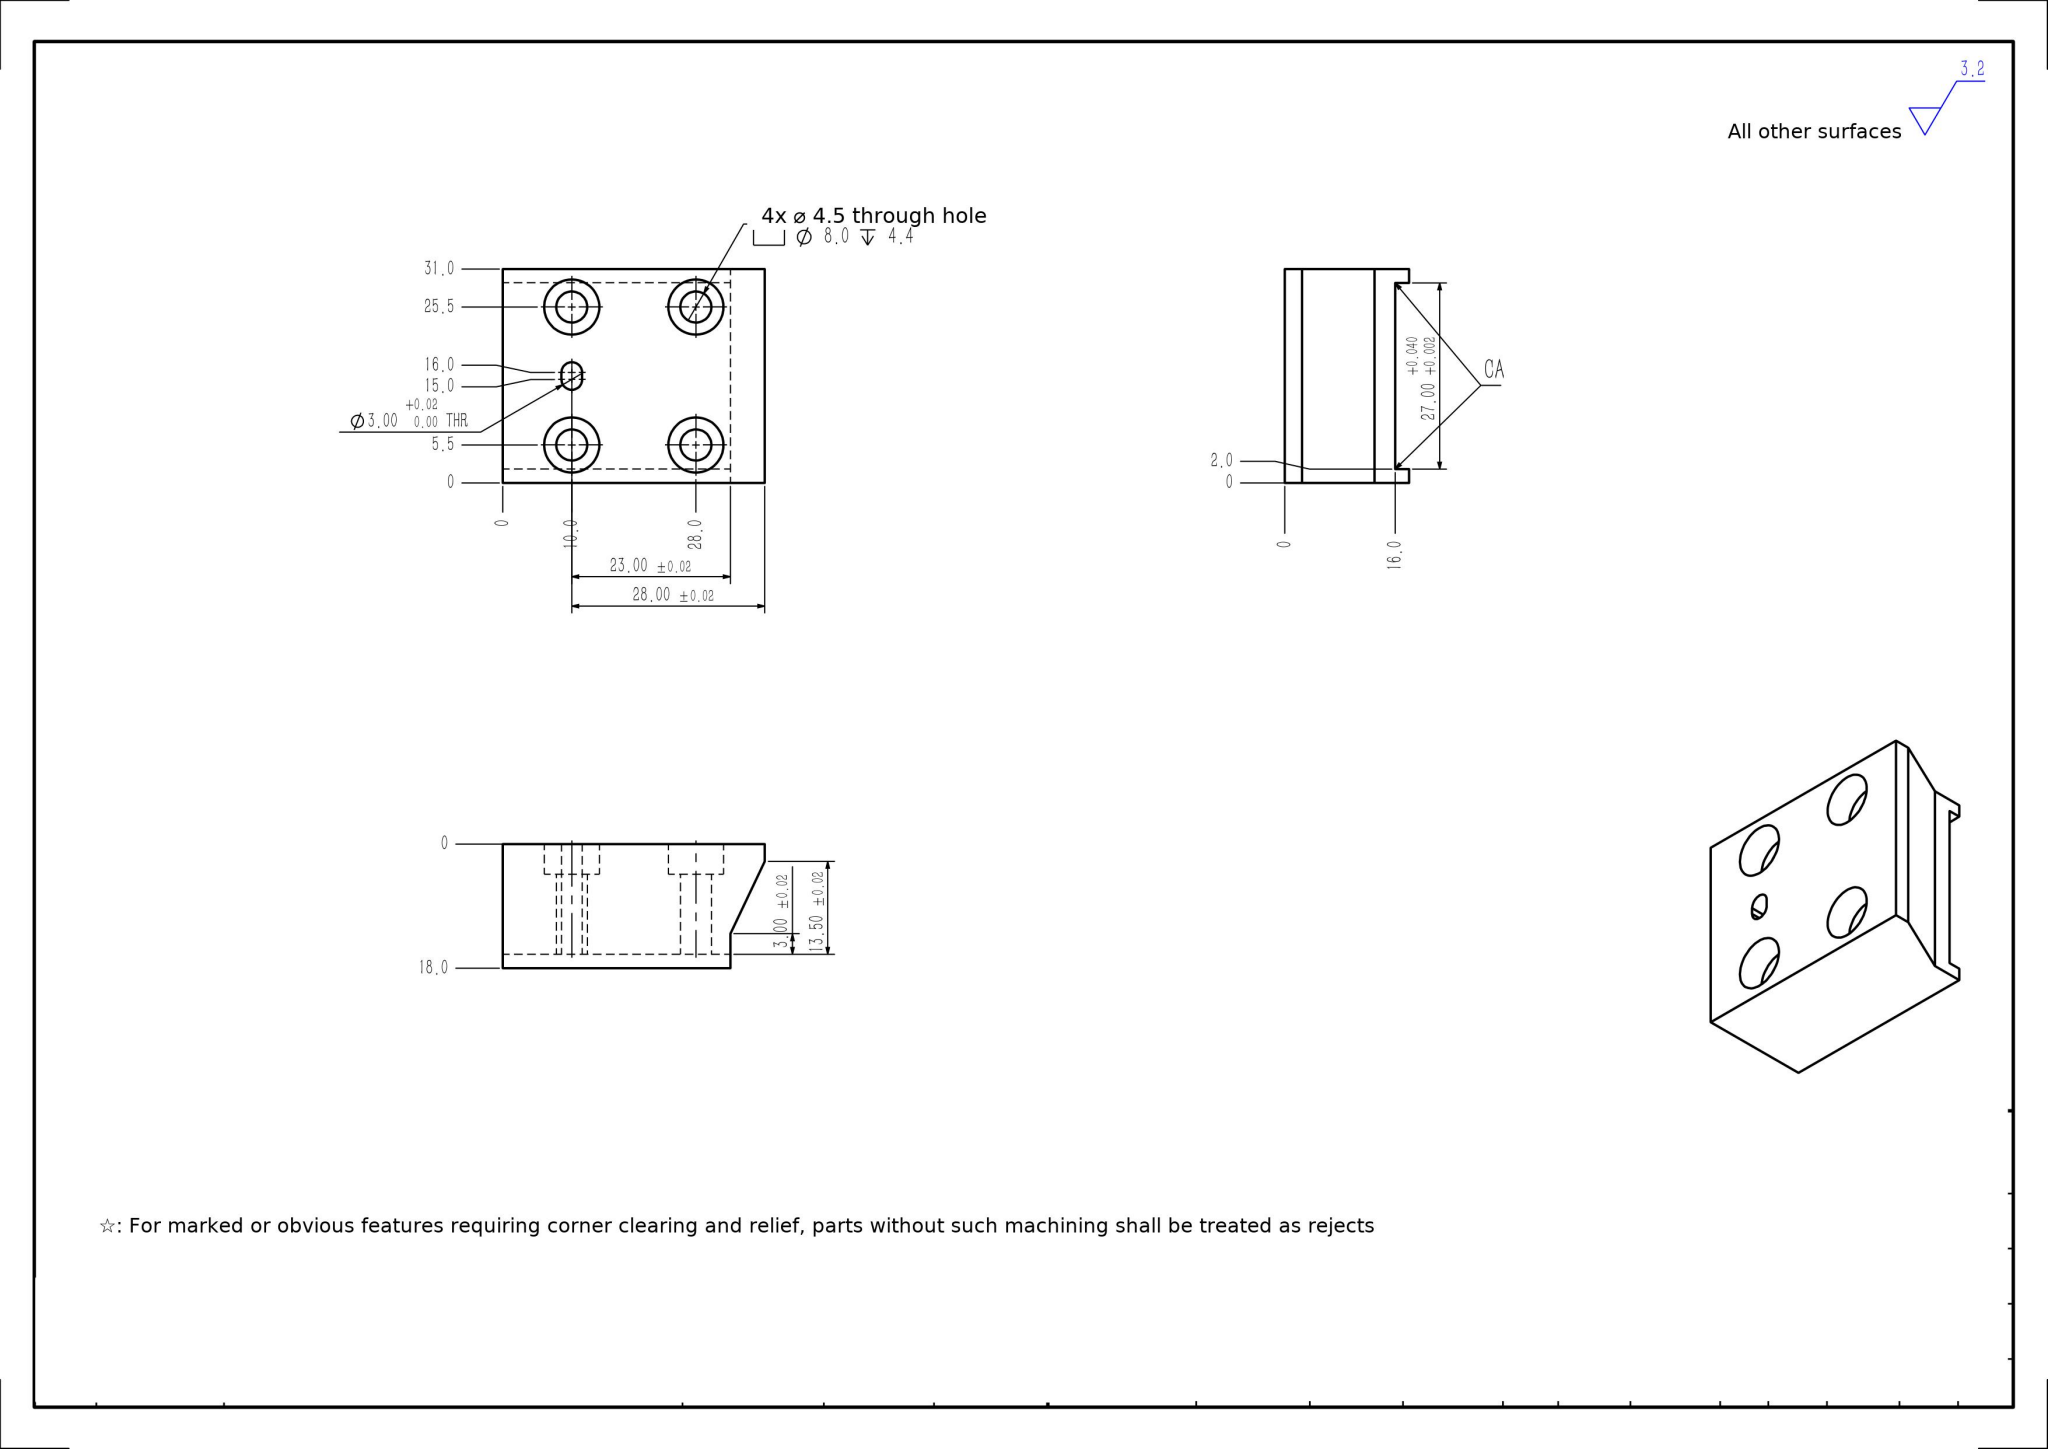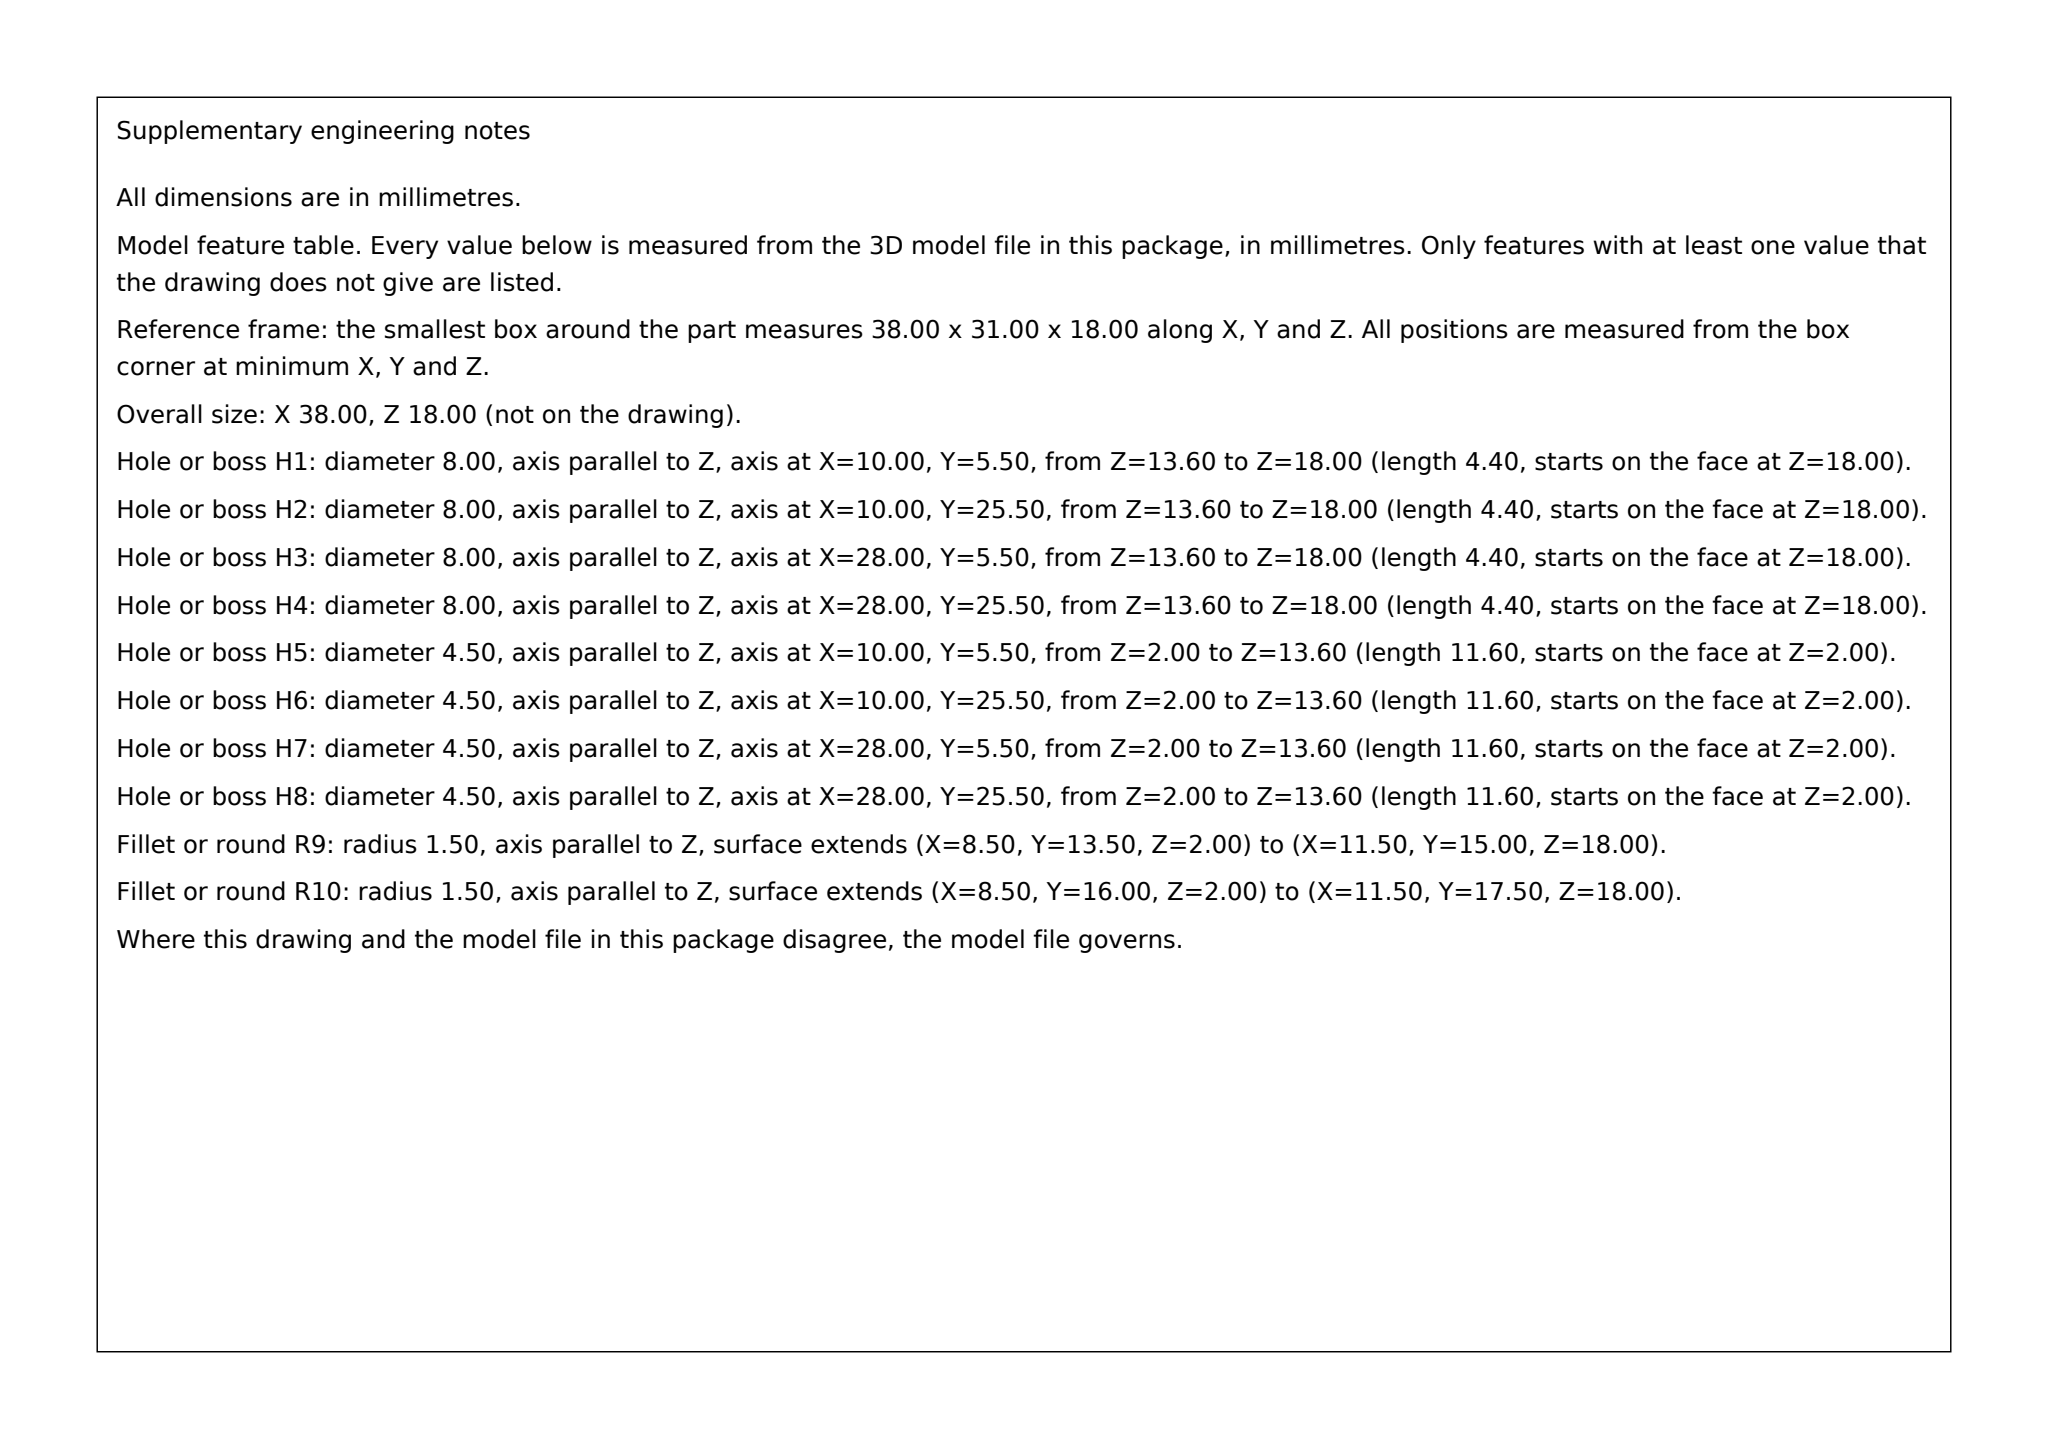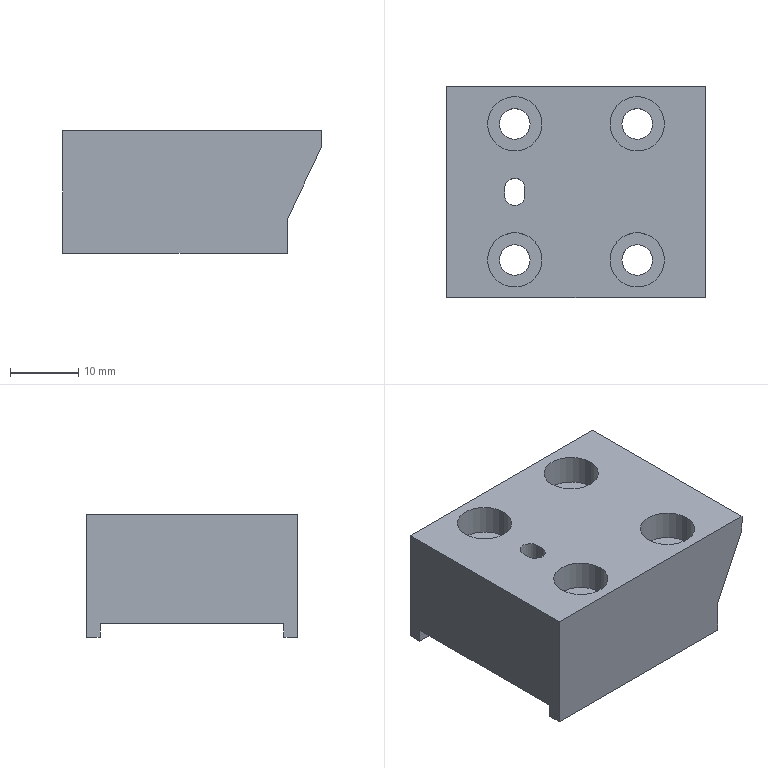Part | SolidWorks | mm | 1 solid | 36 faces | box 38 x 31 x 18 mm | volume 16050 mm3 | cylinder 18 | plane 18 | commonest cylinder face diameters 8 x8 4.5 x8 3 x2
build123d program:
from build123d import *

# Parameters (mm, degrees)
SKETCH1_W                                       = 38
SKETCH1_H                                       = 31
BOSS_EXTRUDE1_DEPTH                             = 18
SKETCH2_W                                       = 38
SKETCH2_H                                       = 27
CUT_EXTRUDE1_DEPTH                              = 2
M4_HEX_SOCKET_HEAD_CAP_SCREW_CBORE1_D           = 4.5
M4_HEX_SOCKET_HEAD_CAP_SCREW_CBORE1_CBORE_D     = 8
M4_HEX_SOCKET_HEAD_CAP_SCREW_CBORE1_CBORE_DEPTH = 4.4
SIZE_MM_DOWEL_PIN_HOLE_1_D                      = 3
CUT_EXTRUDE7_DEPTH                              = 41.571
CUT_EXTRUDE8_DEPTH                              = 31.418


with BuildPart() as part:
    # Sketch1 → Boss-Extrude1 (new body)
    with BuildSketch(Plane.XY):
        Rectangle(SKETCH1_W, SKETCH1_H)
    extrude(amount=BOSS_EXTRUDE1_DEPTH)

    # Sketch2 → Cut-Extrude1 (cut)
    with BuildSketch(Plane(origin=(0, 0, 0), x_dir=(-1, 0, 0), z_dir=(0, 0, -1))):
        Rectangle(SKETCH2_W, SKETCH2_H)
    extrude(amount=-CUT_EXTRUDE1_DEPTH, mode=Mode.SUBTRACT)

    # M4 Hex Socket Head Cap Screw CBORE1 (through all)
    with Locations(Plane.XY.offset(18)):
        with Locations((-9, 10), (9, 10), (-9, -10), (9, -10)):
            CounterBoreHole(M4_HEX_SOCKET_HEAD_CAP_SCREW_CBORE1_D / 2, M4_HEX_SOCKET_HEAD_CAP_SCREW_CBORE1_CBORE_D / 2, M4_HEX_SOCKET_HEAD_CAP_SCREW_CBORE1_CBORE_DEPTH)

    # Size mm Dowel Pin Hole 1 (through all)
    with Locations(Plane.XY.offset(18)):
        with Locations((-9, 0)):
            Hole(SIZE_MM_DOWEL_PIN_HOLE_1_D / 2)

    # Sketch14 → Cut-Extrude7 (cut, through all)
    with BuildSketch(Plane(origin=(0, -15.5, 0), x_dir=(-1, 0, 0), z_dir=(0, -1, 0))):
        Polygon((-19, -15.5), (-14, -5), (-14, 0), (-19, 0), align=None)
    extrude(amount=-CUT_EXTRUDE7_DEPTH, mode=Mode.SUBTRACT)

    # Sketch15 → Cut-Extrude8 (cut, through all)
    with BuildSketch(Plane.XY.offset(18)):
        with BuildLine():
            Line((-10.5, -0.5), (-10.5, 0.5))
            ThreePointArc((-10.5, 0.5), (-9, 2), (-7.5, 0.5))
            Line((-7.5, 0.5), (-7.5, -0.5))
            ThreePointArc((-7.5, -0.5), (-9, -2), (-10.5, -0.5))
        make_face()
    extrude(amount=-CUT_EXTRUDE8_DEPTH, mode=Mode.SUBTRACT)


solid = part.part